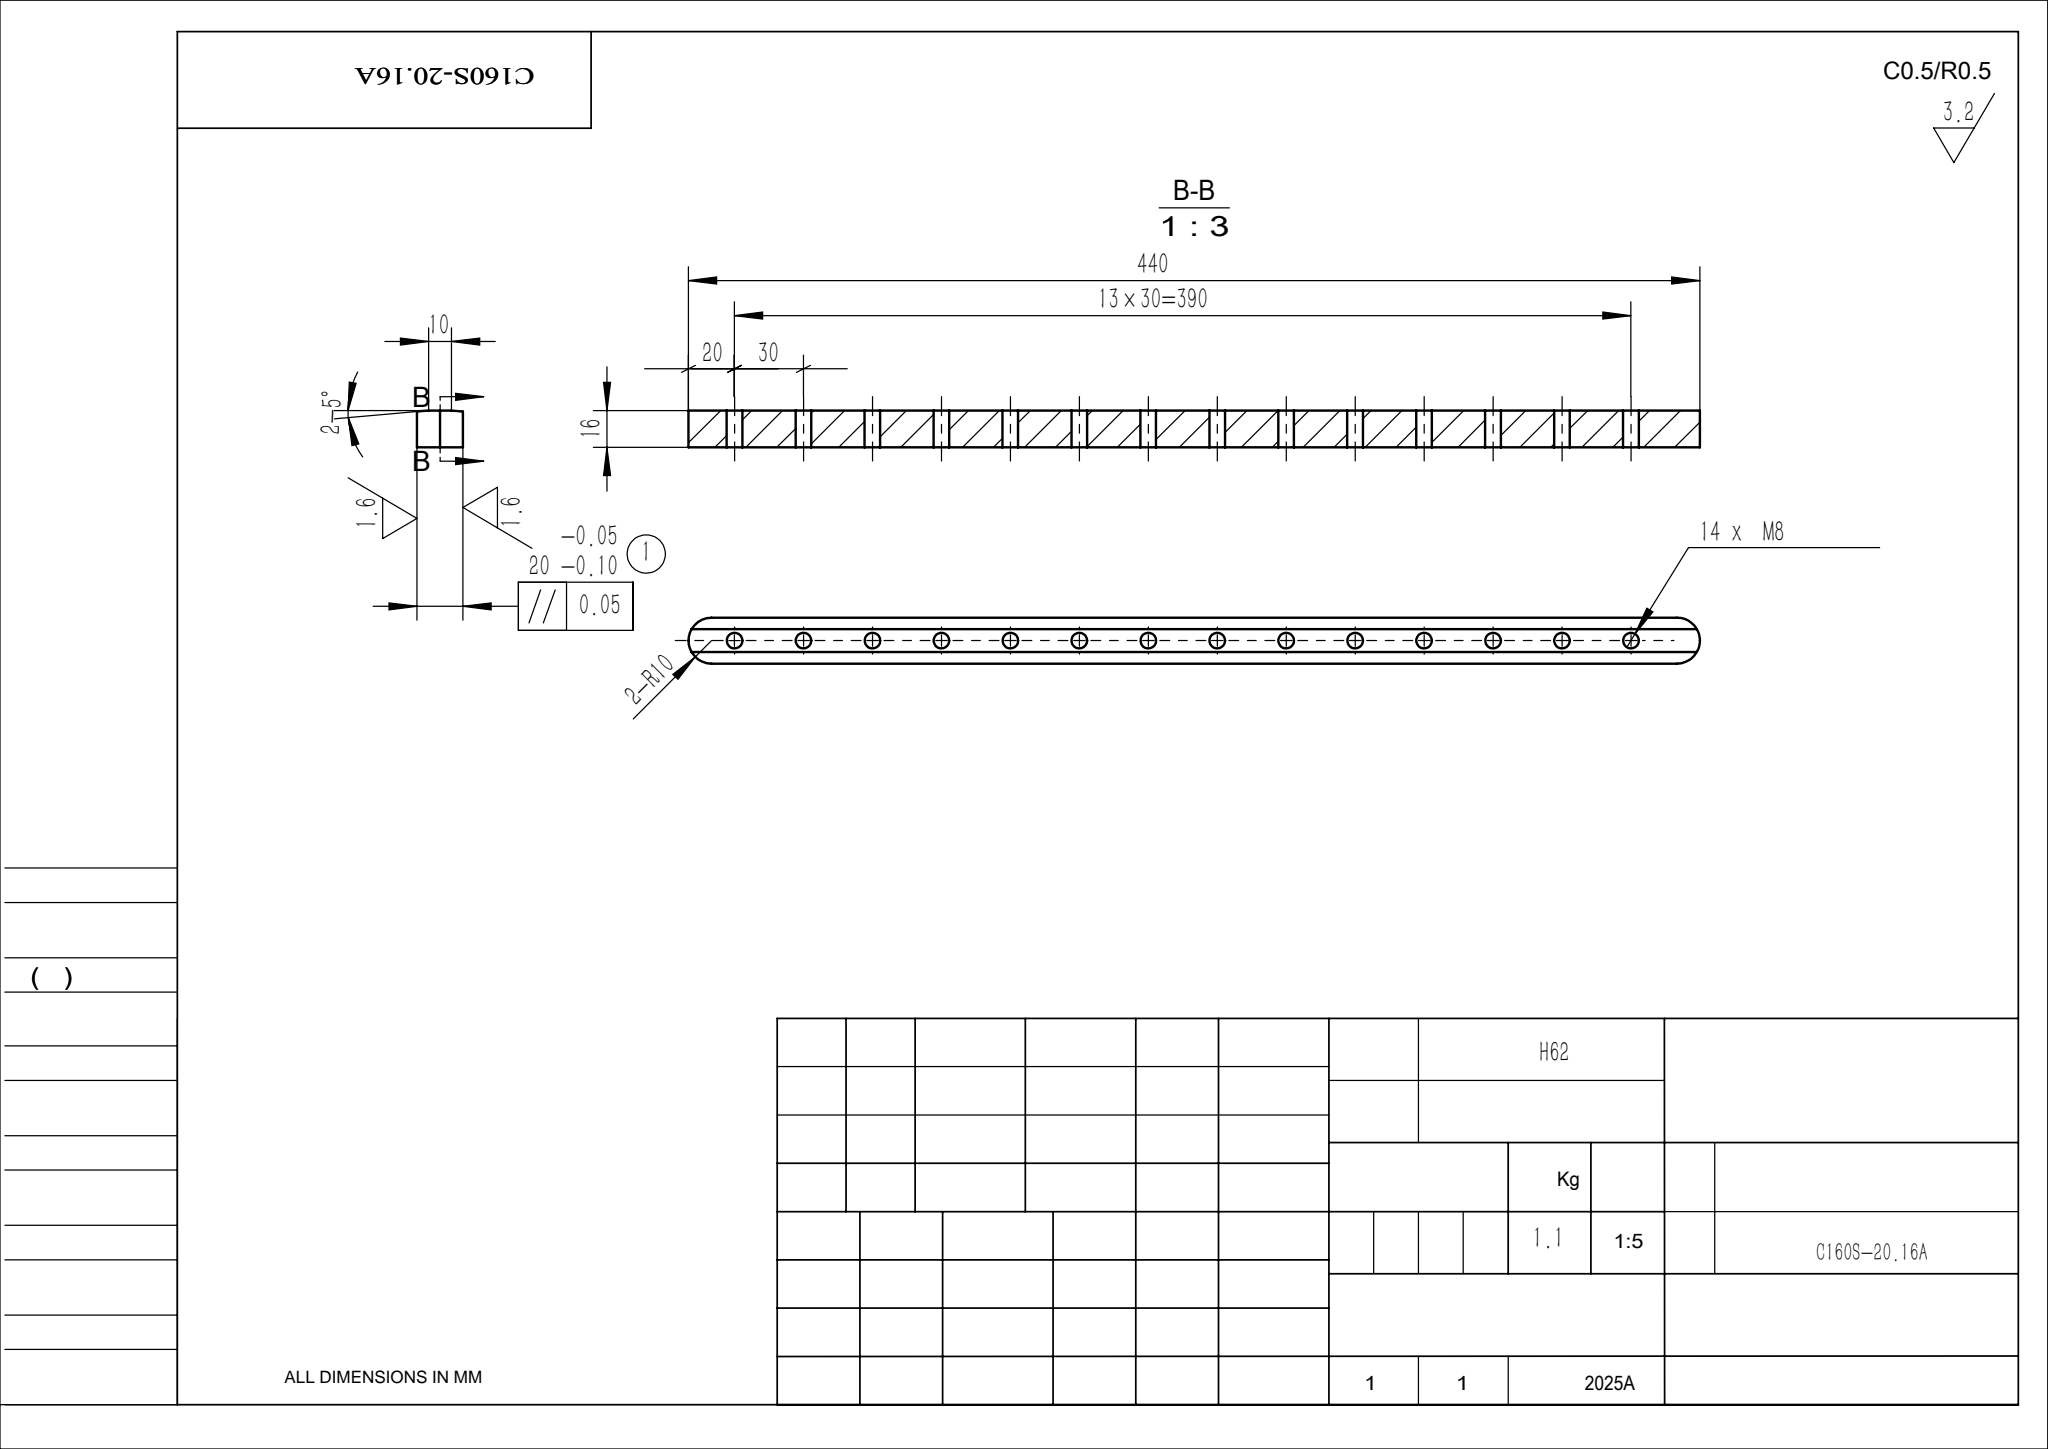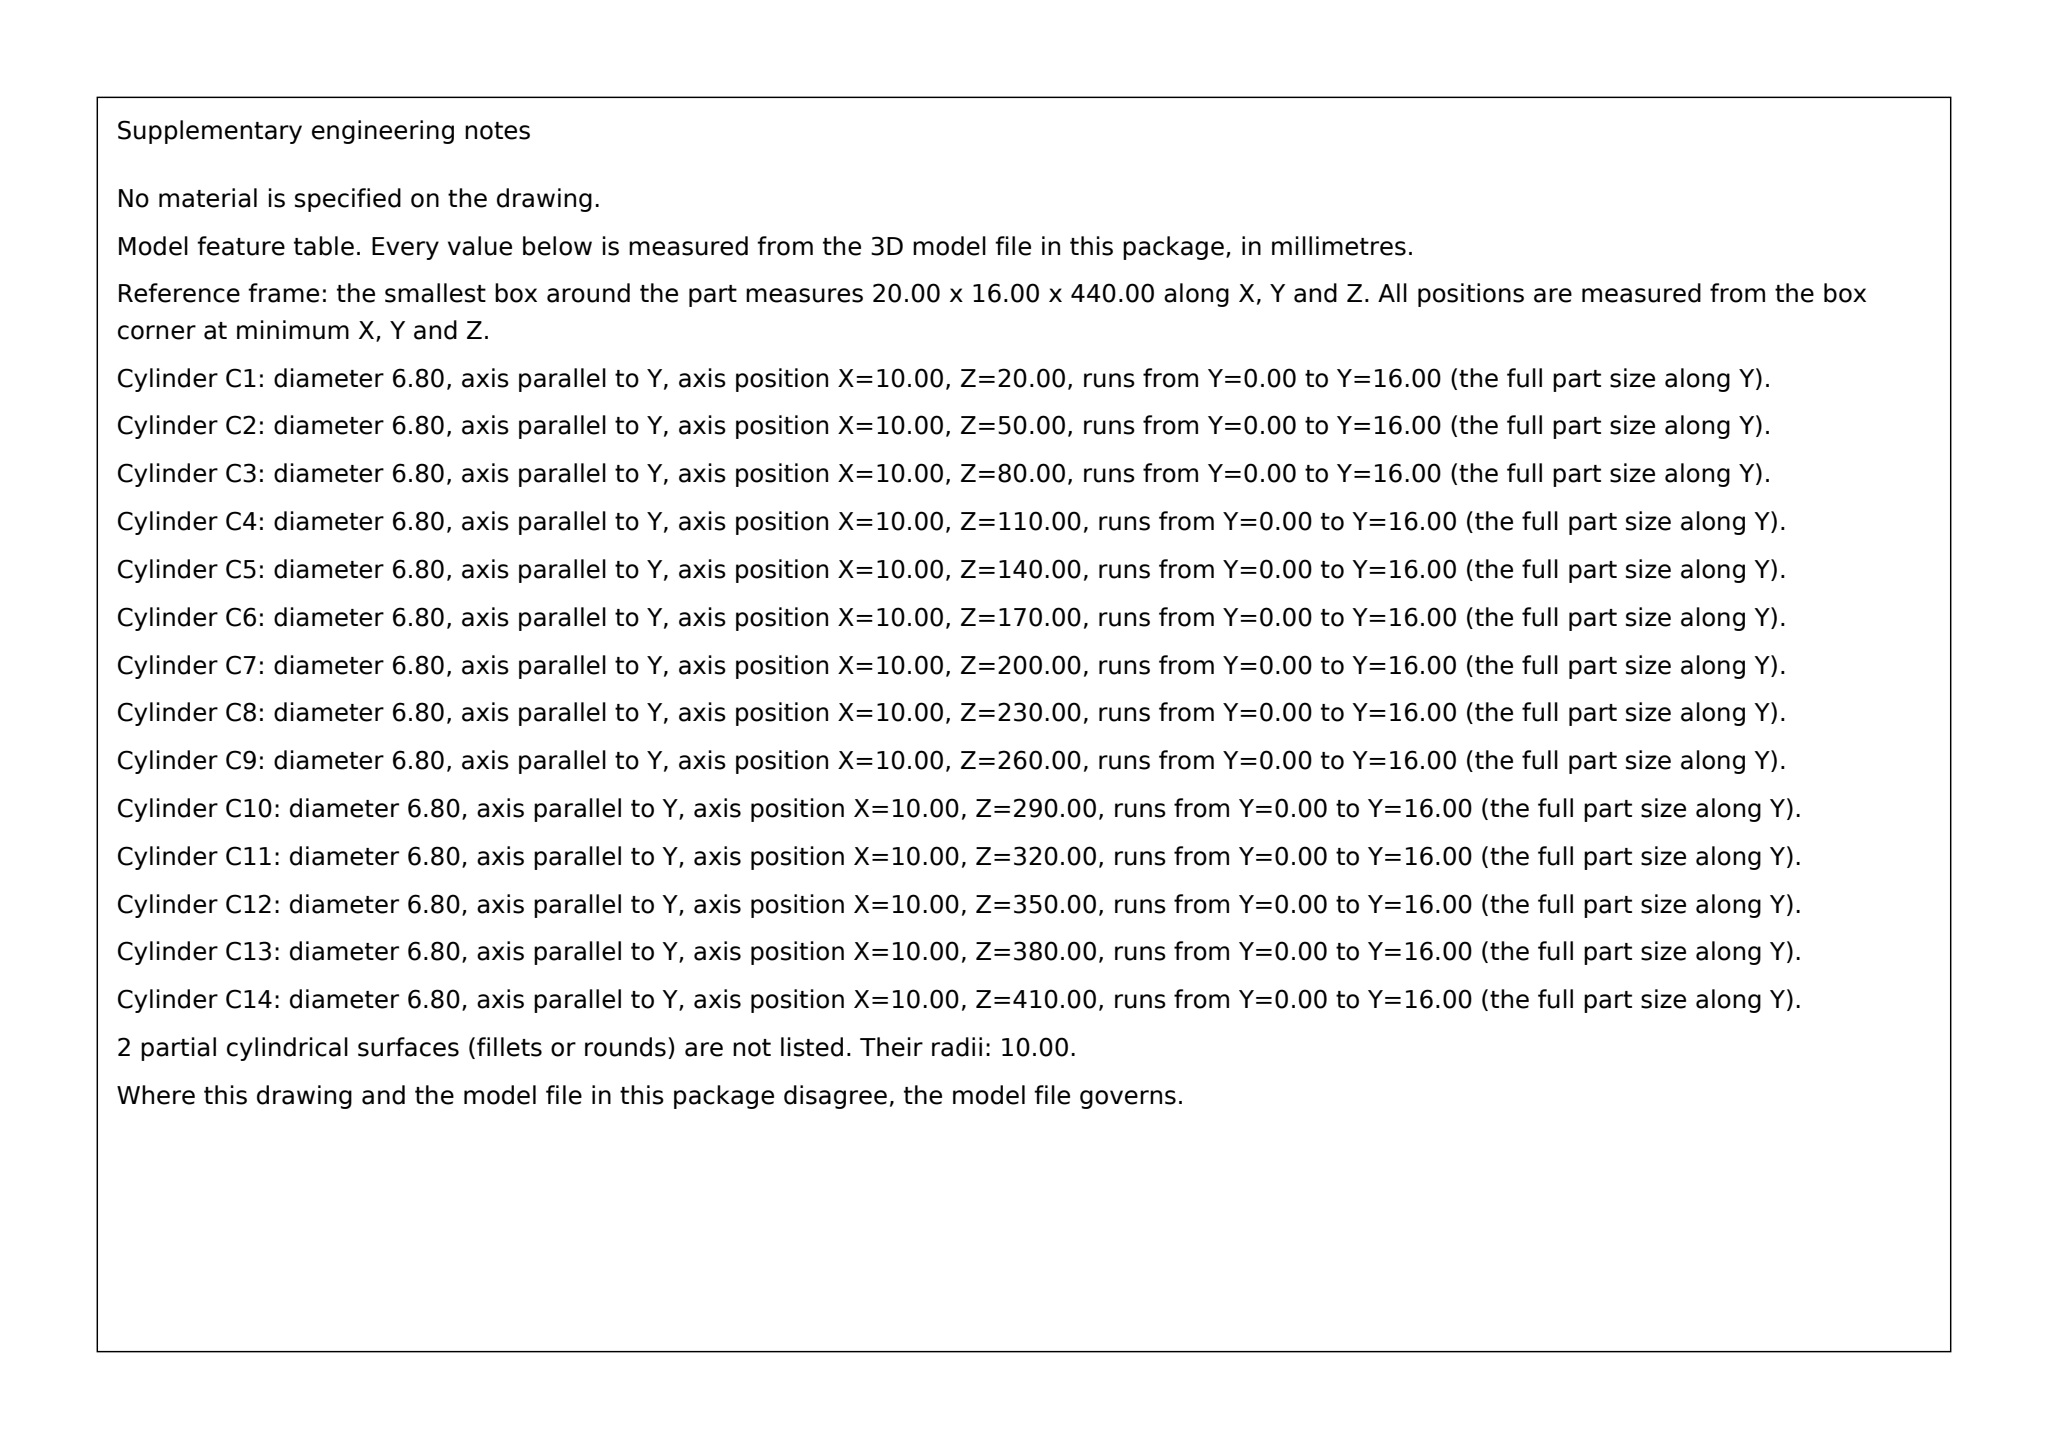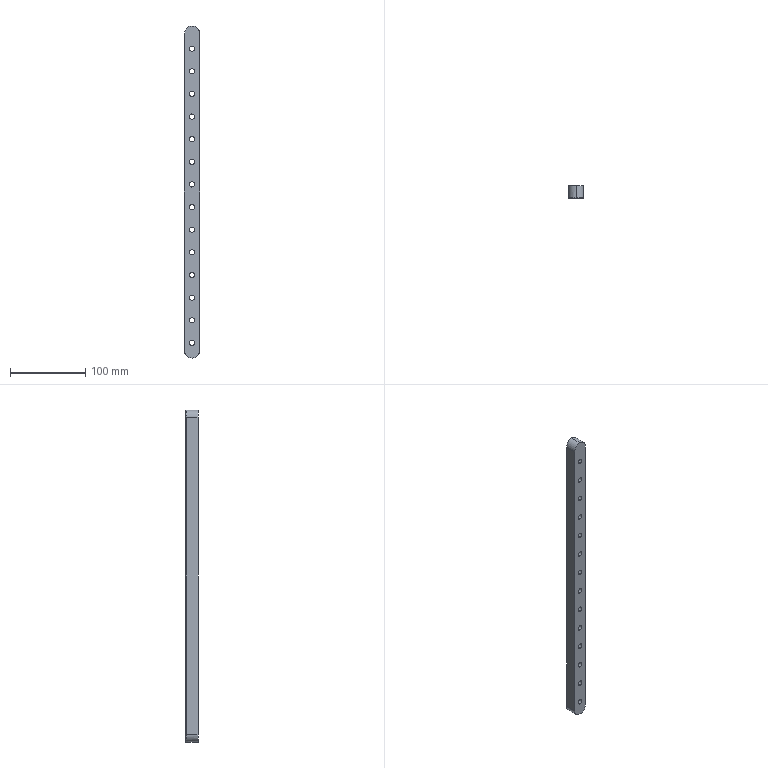Part | SolidWorks | mm | material H62 | 1 solid | 38 faces | box 20 x 16 x 440 mm | volume 130351 mm3 | cylinder 32 | plane 6 | commonest cylinder face diameters 6.8 x28 20 x4